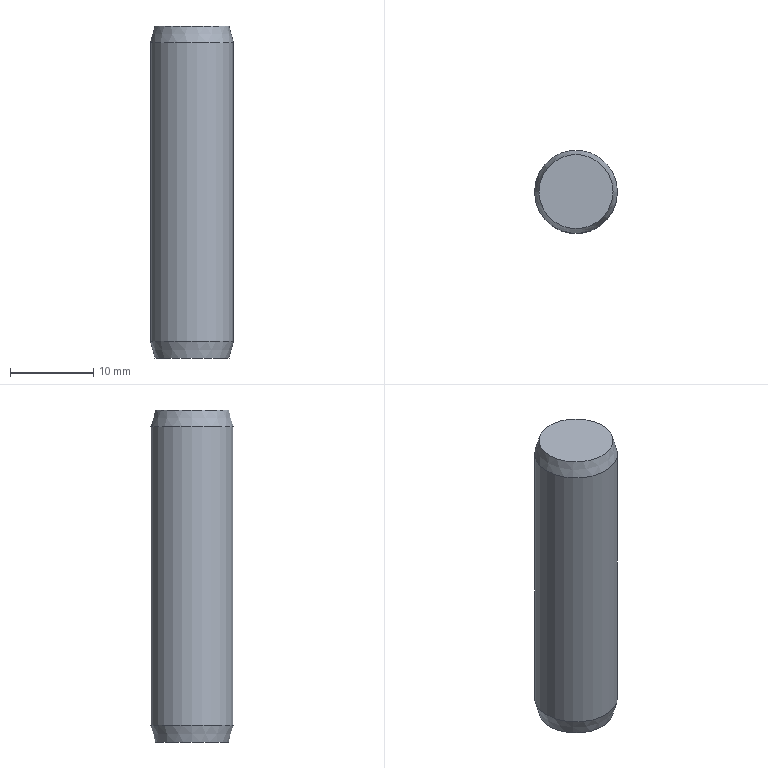Component | NX | GB-T119_1-2000_10X40 | 1 solid | 5 faces | box 10 x 10 x 40 mm | volume 3109 mm3 | plane 2 | cone 2 | cylinder 1 | commonest cylinder face diameters 10 x1
STEP:
#1=CARTESIAN_POINT('',(0.,0.,0.));
#2=DIRECTION('',(0.,0.,1.));
#3=DIRECTION('',(1.,0.,0.));
#4=AXIS2_PLACEMENT_3D('',#1,#2,#3);
#5=CARTESIAN_POINT('',(-202.464,80.,14.));
#6=VERTEX_POINT('',#5);
#7=CARTESIAN_POINT('',(-198.,80.,14.));
#8=DIRECTION('',(0.,0.,-1.));
#9=DIRECTION('',(-1.,0.,0.));
#10=AXIS2_PLACEMENT_3D('',#7,#8,#9);
#11=CIRCLE('',#10,4.464);
#12=CARTESIAN_POINT('',(-198.,80.,14.));
#13=DIRECTION('',(0.,0.,-1.));
#14=DIRECTION('',(-1.,0.,0.));
#15=AXIS2_PLACEMENT_3D('',#12,#13,#14);
#16=PLANE('',#15);
#17=CARTESIAN_POINT('',(0.,0.));
#18=DIRECTION('',(1.,0.));
#19=AXIS2_PLACEMENT_2D('',#17,#18);
#20=CIRCLE('',#19,4.464);
#21=(GEOMETRIC_REPRESENTATION_CONTEXT(2)PARAMETRIC_REPRESENTATION_CONTEXT()REPRESENTATION_CONTEXT('',''));
#22=DEFINITIONAL_REPRESENTATION('',(#20),#21);
#23=PCURVE('',#16,#22);
#24=CARTESIAN_POINT('',(-198.,80.,14.));
#25=DIRECTION('',(0.,0.,1.));
#26=DIRECTION('',(1.,0.,0.));
#27=AXIS2_PLACEMENT_3D('',#24,#25,#26);
#28=CONICAL_SURFACE('',#27,4.464,0.2618);
#29=CARTESIAN_POINT('',(9.425,0.));
#30=DIRECTION('',(-1.,0.));
#31=VECTOR('',#30,1.);
#32=LINE('',#29,#31);
#33=(GEOMETRIC_REPRESENTATION_CONTEXT(2)PARAMETRIC_REPRESENTATION_CONTEXT()REPRESENTATION_CONTEXT('',''));
#34=DEFINITIONAL_REPRESENTATION('',(#32),#33);
#35=PCURVE('',#28,#34);
#36=SURFACE_CURVE('',#11,(#23,#35),.PCURVE_S1.);
#37=EDGE_CURVE('',#6,#6,#36,.T.);
#38=ORIENTED_EDGE('',*,*,#37,.T.);
#39=EDGE_LOOP('',(#38));
#40=FACE_BOUND('',#39,.T.);
#41=ADVANCED_FACE('',(#40),#16,.T.);
#42=CARTESIAN_POINT('',(-203.,80.,16.));
#43=VERTEX_POINT('',#42);
#44=CARTESIAN_POINT('',(-198.,80.,16.));
#45=DIRECTION('',(0.,0.,-1.));
#46=DIRECTION('',(-1.,0.,0.));
#47=AXIS2_PLACEMENT_3D('',#44,#45,#46);
#48=CIRCLE('',#47,5.);
#49=CARTESIAN_POINT('',(9.425,2.));
#50=DIRECTION('',(-1.,0.));
#51=VECTOR('',#50,1.);
#52=LINE('',#49,#51);
#53=(GEOMETRIC_REPRESENTATION_CONTEXT(2)PARAMETRIC_REPRESENTATION_CONTEXT()REPRESENTATION_CONTEXT('',''));
#54=DEFINITIONAL_REPRESENTATION('',(#52),#53);
#55=PCURVE('',#28,#54);
#56=CARTESIAN_POINT('',(-198.,80.,54.));
#57=DIRECTION('',(0.,0.,-1.));
#58=DIRECTION('',(-1.,0.,0.));
#59=AXIS2_PLACEMENT_3D('',#56,#57,#58);
#60=CYLINDRICAL_SURFACE('',#59,5.);
#61=CARTESIAN_POINT('',(0.,38.));
#62=DIRECTION('',(1.,0.));
#63=VECTOR('',#62,1.);
#64=LINE('',#61,#63);
#65=(GEOMETRIC_REPRESENTATION_CONTEXT(2)PARAMETRIC_REPRESENTATION_CONTEXT()REPRESENTATION_CONTEXT('',''));
#66=DEFINITIONAL_REPRESENTATION('',(#64),#65);
#67=PCURVE('',#60,#66);
#68=SURFACE_CURVE('',#48,(#55,#67),.PCURVE_S1.);
#69=EDGE_CURVE('',#43,#43,#68,.T.);
#70=ORIENTED_EDGE('',*,*,#69,.T.);
#71=CARTESIAN_POINT('',(-202.464,80.,14.));
#72=CARTESIAN_POINT('',(-203.,80.,16.));
#73=B_SPLINE_CURVE_WITH_KNOTS('',1,(#71,#72),.UNSPECIFIED.,.F.,.F.,(2,2),(0.,2.071),.PIECEWISE_BEZIER_KNOTS.);
#74=CARTESIAN_POINT('',(3.142,0.));
#75=DIRECTION('',(0.,1.));
#76=VECTOR('',#75,1.);
#77=LINE('',#74,#76);
#78=(GEOMETRIC_REPRESENTATION_CONTEXT(2)PARAMETRIC_REPRESENTATION_CONTEXT()REPRESENTATION_CONTEXT('',''));
#79=DEFINITIONAL_REPRESENTATION('',(#77),#78);
#80=PCURVE('',#28,#79);
#81=CARTESIAN_POINT('',(9.425,0.));
#82=DIRECTION('',(0.,1.));
#83=VECTOR('',#82,1.);
#84=LINE('',#81,#83);
#85=(GEOMETRIC_REPRESENTATION_CONTEXT(2)PARAMETRIC_REPRESENTATION_CONTEXT()REPRESENTATION_CONTEXT('',''));
#86=DEFINITIONAL_REPRESENTATION('',(#84),#85);
#87=PCURVE('',#28,#86);
#88=SEAM_CURVE('',#73,(#80,#87),.PCURVE_S1.);
#89=EDGE_CURVE('',#6,#43,#88,.T.);
#90=ORIENTED_EDGE('',*,*,#89,.F.);
#91=ORIENTED_EDGE('',*,*,#37,.F.);
#92=ORIENTED_EDGE('',*,*,#89,.T.);
#93=EDGE_LOOP('',(#70,#90,#91,#92));
#94=FACE_BOUND('',#93,.T.);
#95=ADVANCED_FACE('',(#94),#28,.T.);
#96=CARTESIAN_POINT('',(-203.,80.,52.));
#97=VERTEX_POINT('',#96);
#98=CARTESIAN_POINT('',(-198.,80.,52.));
#99=DIRECTION('',(0.,0.,-1.));
#100=DIRECTION('',(-1.,0.,0.));
#101=AXIS2_PLACEMENT_3D('',#98,#99,#100);
#102=CIRCLE('',#101,5.);
#103=CARTESIAN_POINT('',(0.,2.));
#104=DIRECTION('',(1.,0.));
#105=VECTOR('',#104,1.);
#106=LINE('',#103,#105);
#107=(GEOMETRIC_REPRESENTATION_CONTEXT(2)PARAMETRIC_REPRESENTATION_CONTEXT()REPRESENTATION_CONTEXT('',''));
#108=DEFINITIONAL_REPRESENTATION('',(#106),#107);
#109=PCURVE('',#60,#108);
#110=CARTESIAN_POINT('',(-198.,80.,52.));
#111=DIRECTION('',(0.,0.,-1.));
#112=DIRECTION('',(-1.,0.,0.));
#113=AXIS2_PLACEMENT_3D('',#110,#111,#112);
#114=CONICAL_SURFACE('',#113,5.,0.2618);
#115=CARTESIAN_POINT('',(0.,0.));
#116=DIRECTION('',(1.,0.));
#117=VECTOR('',#116,1.);
#118=LINE('',#115,#117);
#119=(GEOMETRIC_REPRESENTATION_CONTEXT(2)PARAMETRIC_REPRESENTATION_CONTEXT()REPRESENTATION_CONTEXT('',''));
#120=DEFINITIONAL_REPRESENTATION('',(#118),#119);
#121=PCURVE('',#114,#120);
#122=SURFACE_CURVE('',#102,(#109,#121),.PCURVE_S1.);
#123=EDGE_CURVE('',#97,#97,#122,.T.);
#124=ORIENTED_EDGE('',*,*,#123,.T.);
#125=CARTESIAN_POINT('',(-203.,80.,52.));
#126=CARTESIAN_POINT('',(-203.,80.,16.));
#127=B_SPLINE_CURVE_WITH_KNOTS('',1,(#125,#126),.UNSPECIFIED.,.F.,.F.,(2,2),(2.,38.),.PIECEWISE_BEZIER_KNOTS.);
#128=CARTESIAN_POINT('',(6.283,0.));
#129=DIRECTION('',(0.,1.));
#130=VECTOR('',#129,1.);
#131=LINE('',#128,#130);
#132=(GEOMETRIC_REPRESENTATION_CONTEXT(2)PARAMETRIC_REPRESENTATION_CONTEXT()REPRESENTATION_CONTEXT('',''));
#133=DEFINITIONAL_REPRESENTATION('',(#131),#132);
#134=PCURVE('',#60,#133);
#135=CARTESIAN_POINT('',(0.,0.));
#136=DIRECTION('',(0.,1.));
#137=VECTOR('',#136,1.);
#138=LINE('',#135,#137);
#139=(GEOMETRIC_REPRESENTATION_CONTEXT(2)PARAMETRIC_REPRESENTATION_CONTEXT()REPRESENTATION_CONTEXT('',''));
#140=DEFINITIONAL_REPRESENTATION('',(#138),#139);
#141=PCURVE('',#60,#140);
#142=SEAM_CURVE('',#127,(#134,#141),.PCURVE_S1.);
#143=EDGE_CURVE('',#97,#43,#142,.T.);
#144=ORIENTED_EDGE('',*,*,#143,.T.);
#145=ORIENTED_EDGE('',*,*,#69,.F.);
#146=ORIENTED_EDGE('',*,*,#143,.F.);
#147=EDGE_LOOP('',(#124,#144,#145,#146));
#148=FACE_BOUND('',#147,.T.);
#149=ADVANCED_FACE('',(#148),#60,.T.);
#150=CARTESIAN_POINT('',(-202.464,80.,54.));
#151=VERTEX_POINT('',#150);
#152=CARTESIAN_POINT('',(-198.,80.,54.));
#153=DIRECTION('',(0.,0.,-1.));
#154=DIRECTION('',(-1.,0.,0.));
#155=AXIS2_PLACEMENT_3D('',#152,#153,#154);
#156=CIRCLE('',#155,4.464);
#157=CARTESIAN_POINT('',(0.,-2.));
#158=DIRECTION('',(1.,0.));
#159=VECTOR('',#158,1.);
#160=LINE('',#157,#159);
#161=(GEOMETRIC_REPRESENTATION_CONTEXT(2)PARAMETRIC_REPRESENTATION_CONTEXT()REPRESENTATION_CONTEXT('',''));
#162=DEFINITIONAL_REPRESENTATION('',(#160),#161);
#163=PCURVE('',#114,#162);
#164=CARTESIAN_POINT('',(-193.536,80.,54.));
#165=DIRECTION('',(0.,0.,1.));
#166=DIRECTION('',(1.,0.,0.));
#167=AXIS2_PLACEMENT_3D('',#164,#165,#166);
#168=PLANE('',#167);
#169=CARTESIAN_POINT('',(-8.928,0.));
#170=CARTESIAN_POINT('',(-8.928,7.732));
#171=CARTESIAN_POINT('',(-2.232,3.866));
#172=CARTESIAN_POINT('',(4.464,0.));
#173=CARTESIAN_POINT('',(-2.232,-3.866));
#174=CARTESIAN_POINT('',(-8.928,-7.732));
#175=CARTESIAN_POINT('',(-8.928,0.));
#176=(BOUNDED_CURVE()B_SPLINE_CURVE(2,(#169,#170,#171,#172,#173,#174,#175),.UNSPECIFIED.,.T.,.F.)B_SPLINE_CURVE_WITH_KNOTS((1,2,2,2,2,1),(-2.094,0.,2.094,4.189,6.283,8.378),.UNSPECIFIED.)CURVE()GEOMETRIC_REPRESENTATION_ITEM()RATIONAL_B_SPLINE_CURVE((1.,0.5,1.,0.5,1.,0.5,1.))REPRESENTATION_ITEM(''));
#177=(GEOMETRIC_REPRESENTATION_CONTEXT(2)PARAMETRIC_REPRESENTATION_CONTEXT()REPRESENTATION_CONTEXT('',''));
#178=DEFINITIONAL_REPRESENTATION('',(#176),#177);
#179=PCURVE('',#168,#178);
#180=SURFACE_CURVE('',#156,(#163,#179),.PCURVE_S1.);
#181=EDGE_CURVE('',#151,#151,#180,.T.);
#182=ORIENTED_EDGE('',*,*,#181,.T.);
#183=CARTESIAN_POINT('',(-202.464,80.,54.));
#184=CARTESIAN_POINT('',(-203.,80.,52.));
#185=B_SPLINE_CURVE_WITH_KNOTS('',1,(#183,#184),.UNSPECIFIED.,.F.,.F.,(2,2),(-2.071,0.),.PIECEWISE_BEZIER_KNOTS.);
#186=CARTESIAN_POINT('',(6.283,0.));
#187=DIRECTION('',(0.,1.));
#188=VECTOR('',#187,1.);
#189=LINE('',#186,#188);
#190=(GEOMETRIC_REPRESENTATION_CONTEXT(2)PARAMETRIC_REPRESENTATION_CONTEXT()REPRESENTATION_CONTEXT('',''));
#191=DEFINITIONAL_REPRESENTATION('',(#189),#190);
#192=PCURVE('',#114,#191);
#193=CARTESIAN_POINT('',(0.,0.));
#194=DIRECTION('',(0.,1.));
#195=VECTOR('',#194,1.);
#196=LINE('',#193,#195);
#197=(GEOMETRIC_REPRESENTATION_CONTEXT(2)PARAMETRIC_REPRESENTATION_CONTEXT()REPRESENTATION_CONTEXT('',''));
#198=DEFINITIONAL_REPRESENTATION('',(#196),#197);
#199=PCURVE('',#114,#198);
#200=SEAM_CURVE('',#185,(#192,#199),.PCURVE_S1.);
#201=EDGE_CURVE('',#151,#97,#200,.T.);
#202=ORIENTED_EDGE('',*,*,#201,.T.);
#203=ORIENTED_EDGE('',*,*,#123,.F.);
#204=ORIENTED_EDGE('',*,*,#201,.F.);
#205=EDGE_LOOP('',(#182,#202,#203,#204));
#206=FACE_BOUND('',#205,.T.);
#207=ADVANCED_FACE('',(#206),#114,.T.);
#208=ORIENTED_EDGE('',*,*,#181,.F.);
#209=EDGE_LOOP('',(#208));
#210=FACE_BOUND('',#209,.T.);
#211=ADVANCED_FACE('',(#210),#168,.T.);
#212=CLOSED_SHELL('',(#41,#95,#149,#207,#211));
#213=MANIFOLD_SOLID_BREP('',#212);
#214=(LENGTH_UNIT()NAMED_UNIT(*)SI_UNIT(.MILLI.,.METRE.));
#215=UNCERTAINTY_MEASURE_WITH_UNIT(LENGTH_MEASURE(0.00001),#214,'','');
#216=(NAMED_UNIT(*)PLANE_ANGLE_UNIT()SI_UNIT($,.RADIAN.));
#217=(NAMED_UNIT(*)SI_UNIT($,.STERADIAN.)SOLID_ANGLE_UNIT());
#218=(GEOMETRIC_REPRESENTATION_CONTEXT(3)GLOBAL_UNCERTAINTY_ASSIGNED_CONTEXT((#215))GLOBAL_UNIT_ASSIGNED_CONTEXT((#214,#216,#217))REPRESENTATION_CONTEXT('',''));
#219=ADVANCED_BREP_SHAPE_REPRESENTATION('',(#4,#213),#218);